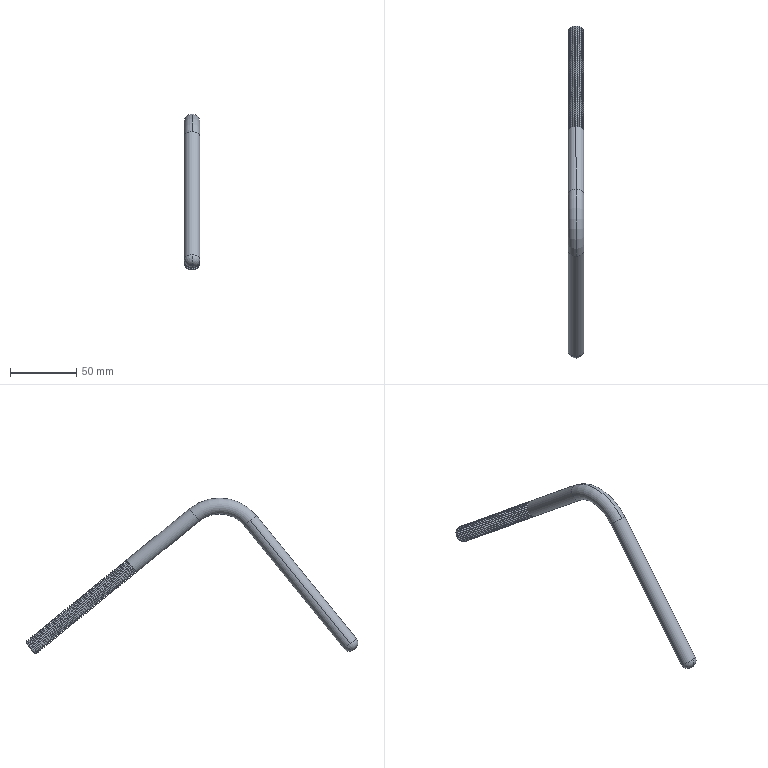Component | SolidWorks | OT-0100-002(Hook)-1 | 1 solid | 306 faces | box 12 x 251.13 x 117.88 mm | volume 36211 mm3 | cone 198 | cylinder 102 | torus 4 | plane 2 | commonest cylinder face diameters 12 x102 | material AISI 304
build123d program:
from build123d import *

# Parameters (mm, degrees)
SKETCH2_R       = 6
LPATTERN1_COUNT = 50
LPATTERN1_PITCH = 2
FILLET1_R       = 5


with BuildPart() as part:
    # Sweep1: sweep along a path in Sketch1
    with BuildLine(Plane(origin=(0, 0, 0), x_dir=(0, 0, -1), z_dir=(1, 0, 0))) as sweep1_path:
        Line((0, 190), (0, 30))
        ThreePointArc((0, 30), (8.787, 8.787), (30, 0))
        Line((30, 0), (155, 0))
    # Sketch2 → Sweep1 (sweep)
    with BuildSketch(Plane(origin=(0, 190, 0), x_dir=(1, 0, 0), z_dir=(0, 1, 0))):
        Circle(SKETCH2_R)
    sweep(path=sweep1_path.line)

    # Sketch3 → Cut-Revolve1 (revolve, cut)
    with BuildSketch(Plane(origin=(0, 0, 0), x_dir=(0, 0, -1), z_dir=(1, 0, 0))):
        Polygon((-6, 189.375), (-4.917, 190), (-6, 190.625), align=None)
    cut_revolve1 = revolve(axis=Axis((0, 0, 0), (0, 1, 0)), mode=Mode.SUBTRACT)

    # LPattern1: Cut-Revolve1 ×50
    with Locations(*[(0, -i * LPATTERN1_PITCH, 0) for i in range(1, LPATTERN1_COUNT)]):
        add(cut_revolve1, mode=Mode.SUBTRACT)

    # Fillet1
    fillet1_edges = [part.edges().sort_by_distance(p)[0] for p in [
        (-6, 0, -155),
    ]]
    fillet(fillet1_edges, radius=FILLET1_R)


solid = part.part

# Placed as in the assembly
solid = solid.moved(Location((-100, -211.429, 227.948), (-39.097, 0, 0)))